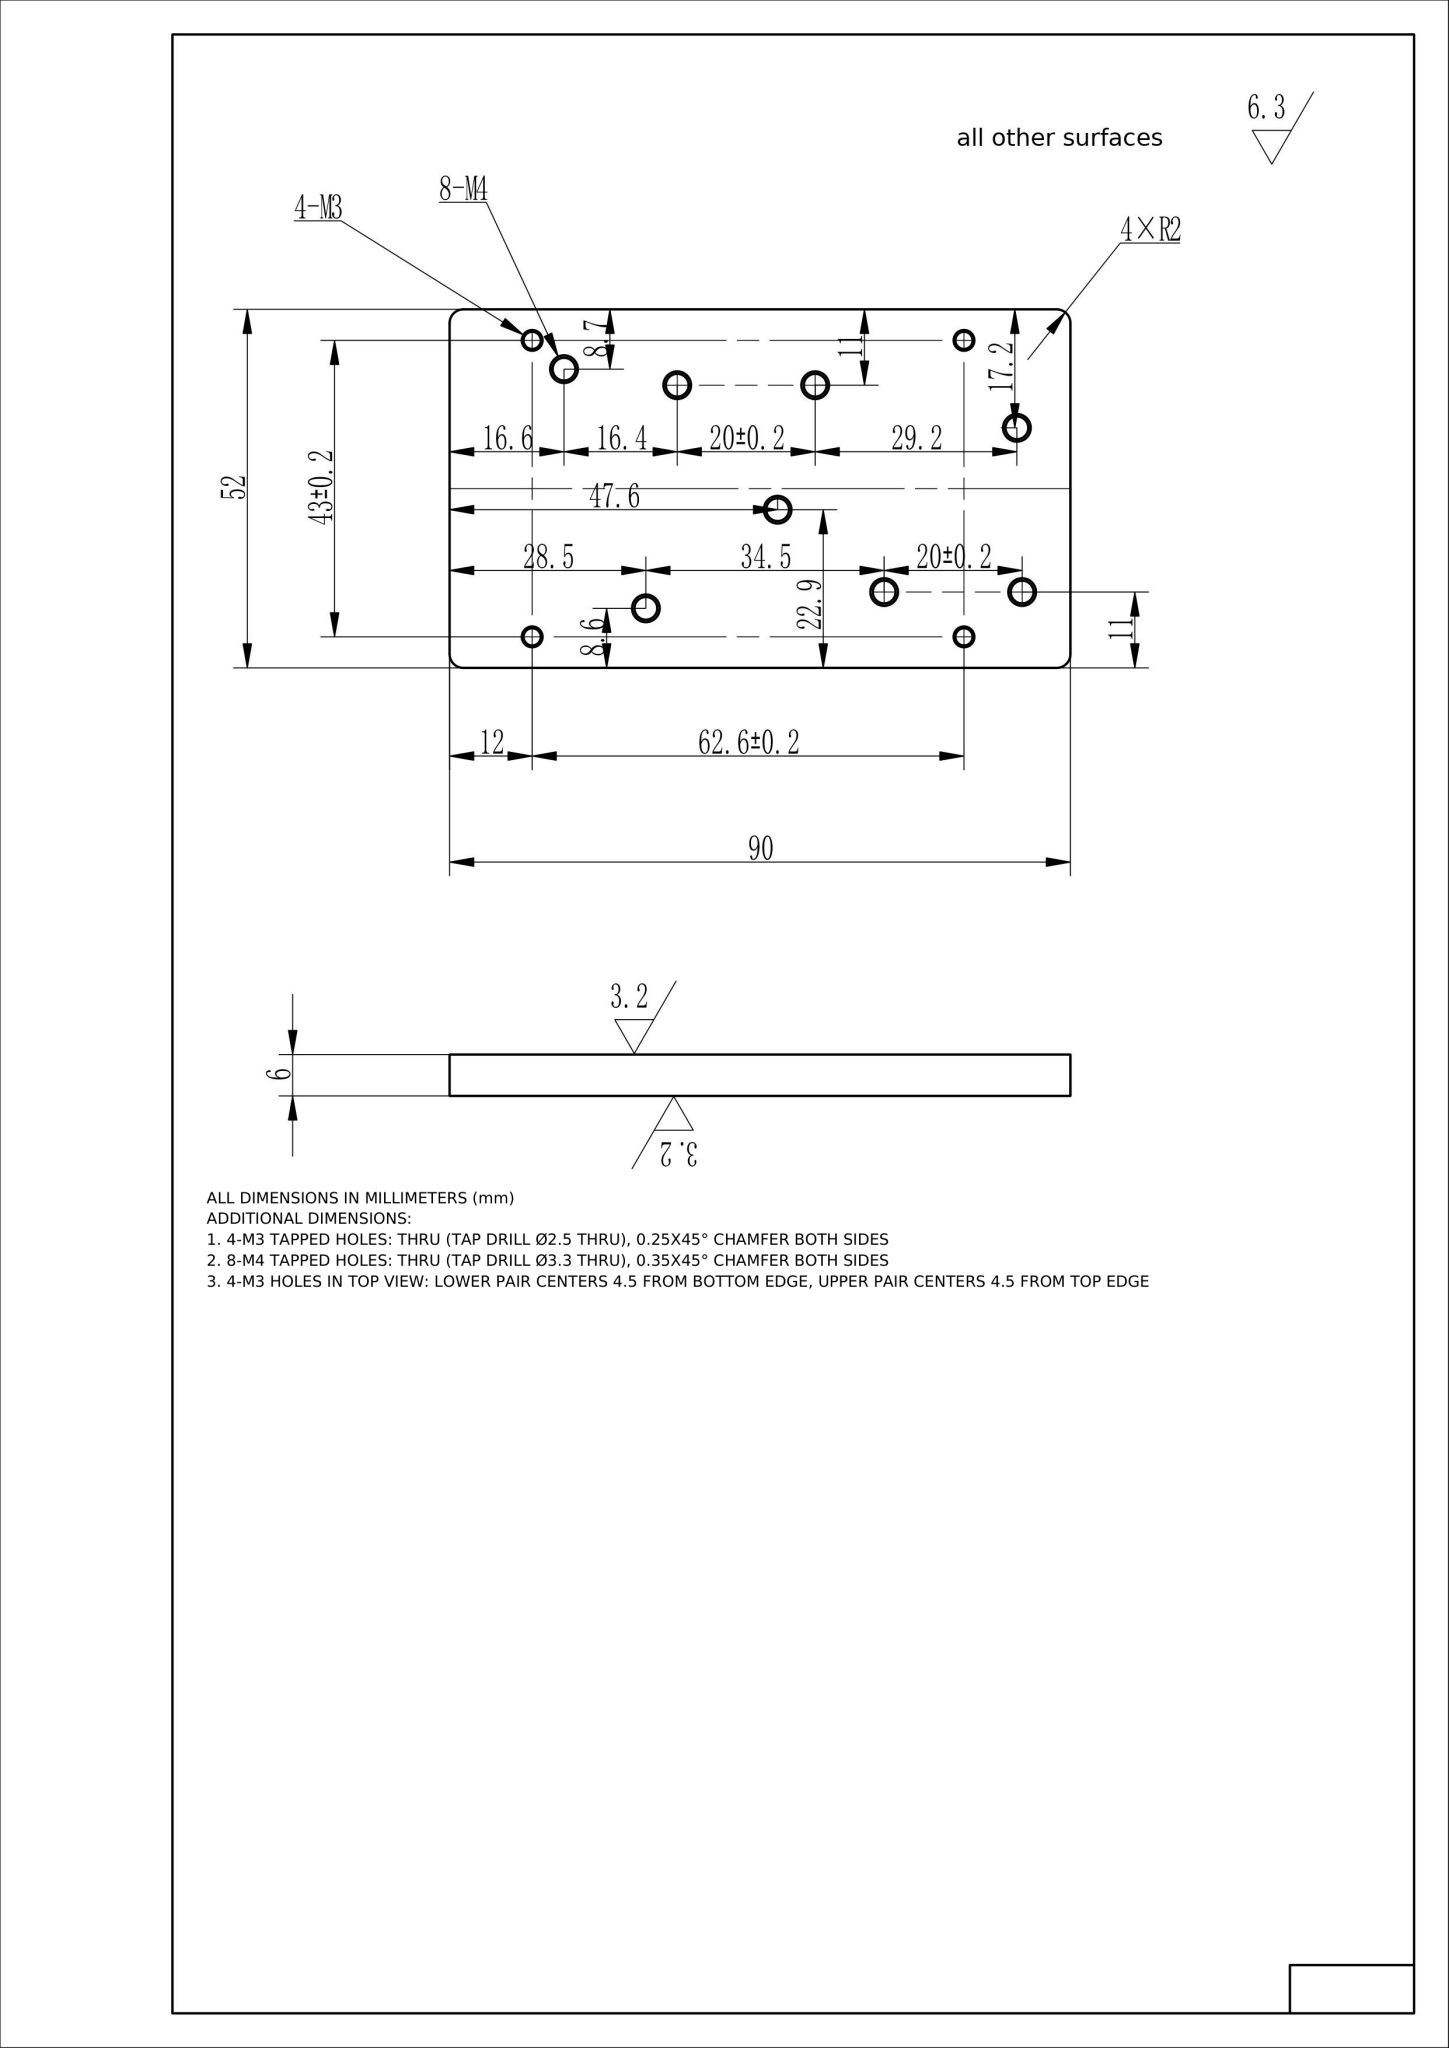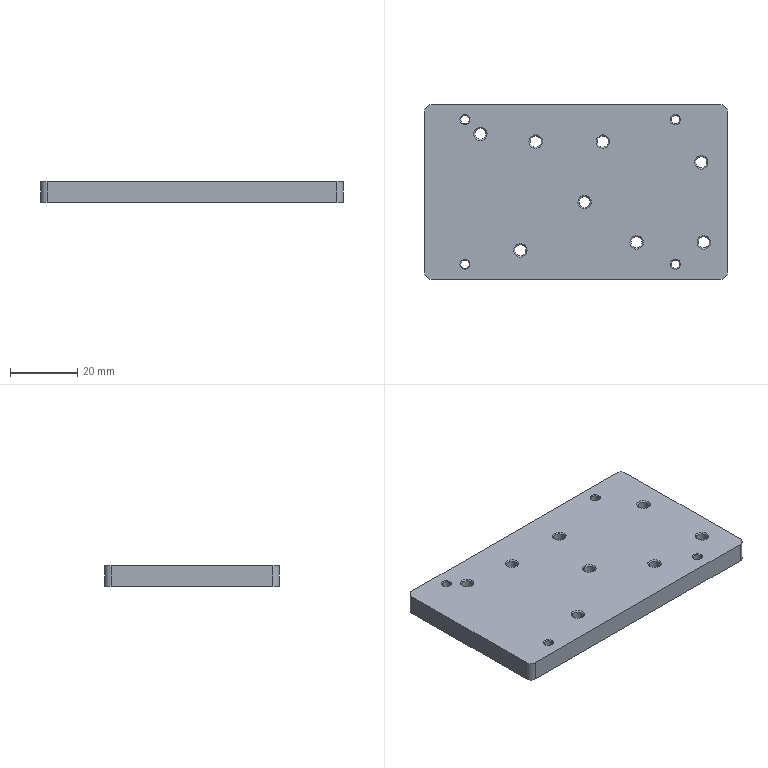Part | NX | mm | 1 solid | 46 faces | box 90 x 52 x 6 mm | volume 27518 mm3 | cone 24 | cylinder 16 | plane 6 | commonest cylinder face diameters 3.3 x8 4 x4 2.5 x4